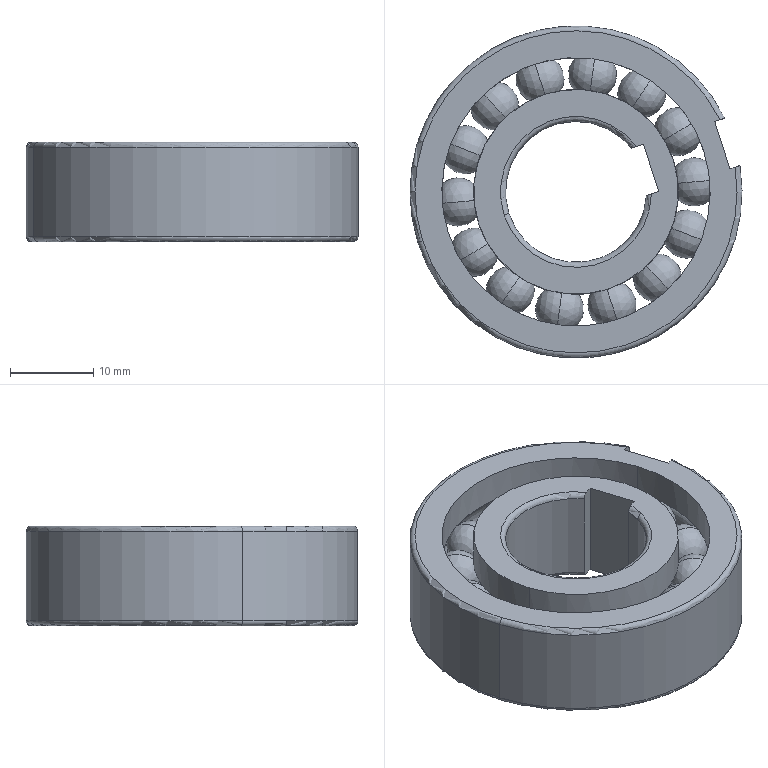Component | SolidWorks | 6203OverrunningBearing0-1 | 1 solid | 103 faces | volume 8941 mm3 | torus 53 | sphere 28 | cylinder 12 | plane 10 | commonest cylinder face diameters 24.67 x4 32.33 x4 17 x2 40 x2 | material GCr15